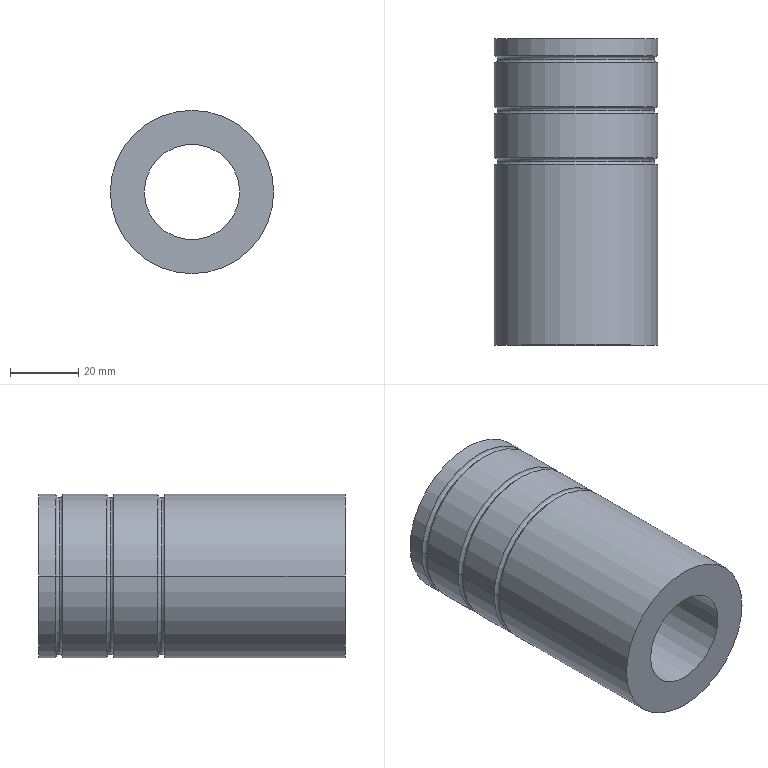Component | SolidWorks | NewDieSet-1_UpperDieSetAssembly-1_GuideBushing-1 | 1 solid | 24 faces | box 48 x 90 x 48 mm | volume 106744 mm3 | torus 12 | cylinder 10 | plane 2 | commonest cylinder face diameters 48 x8 28 x2
build123d program:
from build123d import *

# Parameters (mm, degrees)
SKETCH1_R           = 24
BOSS_EXTRUDE1_DEPTH = 45
SKETCH2_R           = 24
BOSS_EXTRUDE2_DEPTH = 45
SKETCH3_R           = 14
CUT_EXTRUDE1_DEPTH  = 97.187
SKETCH4_R           = 1
LPATTERN1_COUNT     = 3
LPATTERN1_PITCH     = 15


with BuildPart() as part:
    # Sketch1 → Boss-Extrude1 (new body)
    with BuildSketch(Plane.XY):
        with Locations(Location((0, 0, 0), (0, 0, 180))):
            Circle(SKETCH1_R)
    extrude(amount=BOSS_EXTRUDE1_DEPTH)

    # Sketch2 → Boss-Extrude2 (add)
    with BuildSketch(Plane.XY.offset(45)):
        with Locations(Location((0, 0, 0), (0, 0, 180))):
            Circle(SKETCH2_R)
    extrude(amount=BOSS_EXTRUDE2_DEPTH)

    # Sketch3 → Cut-Extrude1 (cut, through all)
    with BuildSketch(Plane.XY.offset(90)):
        Circle(SKETCH3_R)
    extrude(amount=-CUT_EXTRUDE1_DEPTH, mode=Mode.SUBTRACT)

    # Sketch4 → Cut-Revolve1 (revolve, cut)
    with BuildSketch(Plane(origin=(0, 0, 0), x_dir=(1, 0, 0), z_dir=(0, 1, 0)), mode=Mode.PRIVATE) as cut_revolve1_sk:
        with Locations((24, -6)):
            Circle(SKETCH4_R)
    cut_revolve1 = revolve(cut_revolve1_sk.sketch.rotate(Axis((0, 0, 0), (0, 0, 1)), 180), axis=Axis((0, 0, 0), (0, 0, 1)), mode=Mode.SUBTRACT)

    # LPattern1: Cut-Revolve1 ×3
    with Locations(*[(0, 0, i * LPATTERN1_PITCH) for i in range(1, LPATTERN1_COUNT)]):
        add(cut_revolve1, mode=Mode.SUBTRACT)


solid = part.part

# Placed as in the assembly
solid = solid.moved(Location((-216.746, 158.927, 568), (90, 0, 0)))
STEP:
#1=COLOUR_RGB('',0.7922,0.8196,0.9333);
#2=FILL_AREA_STYLE_COLOUR('',#1);
#3=FILL_AREA_STYLE('',(#2));
#4=SURFACE_STYLE_FILL_AREA(#3);
#5=SURFACE_SIDE_STYLE('',(#4));
#6=SURFACE_STYLE_USAGE(.BOTH.,#5);
#7=PRESENTATION_STYLE_ASSIGNMENT((#6));
#8=CARTESIAN_POINT('',(-9.478,4.879,22.362));
#9=VERTEX_POINT('',#8);
#10=CARTESIAN_POINT('',(-9.439,4.84,22.362));
#11=VERTEX_POINT('',#10);
#12=CARTESIAN_POINT('',(-9.478,4.84,22.362));
#13=DIRECTION('',(0.,0.,-1.));
#14=DIRECTION('',(-1.,0.,0.));
#15=AXIS2_PLACEMENT_3D('',#12,#13,#14);
#16=CIRCLE('',#15,0.03937);
#17=EDGE_CURVE('',#9,#11,#16,.T.);
#18=ORIENTED_EDGE('',*,*,#17,.T.);
#19=CARTESIAN_POINT('',(-7.628,4.84,22.362));
#20=VERTEX_POINT('',#19);
#21=CARTESIAN_POINT('',(-8.533,4.84,22.362));
#22=DIRECTION('',(0.,1.,0.));
#23=DIRECTION('',(0.,0.,1.));
#24=AXIS2_PLACEMENT_3D('',#21,#22,#23);
#25=CIRCLE('',#24,0.9055);
#26=EDGE_CURVE('',#11,#20,#25,.T.);
#27=ORIENTED_EDGE('',*,*,#26,.T.);
#28=CARTESIAN_POINT('',(-7.588,4.879,22.362));
#29=VERTEX_POINT('',#28);
#30=CARTESIAN_POINT('',(-7.588,4.84,22.362));
#31=DIRECTION('',(-0.,0.,1.));
#32=DIRECTION('',(1.,0.,0.));
#33=AXIS2_PLACEMENT_3D('',#30,#31,#32);
#34=CIRCLE('',#33,0.03937);
#35=EDGE_CURVE('',#29,#20,#34,.T.);
#36=ORIENTED_EDGE('',*,*,#35,.F.);
#37=CARTESIAN_POINT('',(-8.533,4.879,22.362));
#38=DIRECTION('',(0.,-1.,0.));
#39=DIRECTION('',(1.,0.,0.));
#40=AXIS2_PLACEMENT_3D('',#37,#38,#39);
#41=CIRCLE('',#40,0.9449);
#42=EDGE_CURVE('',#29,#9,#41,.T.);
#43=ORIENTED_EDGE('',*,*,#42,.T.);
#44=EDGE_LOOP('',(#18,#27,#36,#43));
#45=FACE_OUTER_BOUND('',#44,.T.);
#46=CARTESIAN_POINT('',(-8.533,4.84,22.362));
#47=DIRECTION('',(0.,1.,0.));
#48=DIRECTION('',(-1.,0.,0.));
#49=AXIS2_PLACEMENT_3D('',#46,#47,#48);
#50=TOROIDAL_SURFACE('',#49,0.9449,0.03937);
#51=ADVANCED_FACE('',(#45),#50,.F.);
#52=CARTESIAN_POINT('',(-9.478,5.47,22.362));
#53=VERTEX_POINT('',#52);
#54=CARTESIAN_POINT('',(-9.439,5.43,22.362));
#55=VERTEX_POINT('',#54);
#56=CARTESIAN_POINT('',(-9.478,5.43,22.362));
#57=DIRECTION('',(0.,0.,-1.));
#58=DIRECTION('',(-1.,0.,0.));
#59=AXIS2_PLACEMENT_3D('',#56,#57,#58);
#60=CIRCLE('',#59,0.03937);
#61=EDGE_CURVE('',#53,#55,#60,.T.);
#62=ORIENTED_EDGE('',*,*,#61,.T.);
#63=CARTESIAN_POINT('',(-7.628,5.43,22.362));
#64=VERTEX_POINT('',#63);
#65=CARTESIAN_POINT('',(-8.533,5.43,22.362));
#66=DIRECTION('',(0.,1.,0.));
#67=DIRECTION('',(0.,0.,1.));
#68=AXIS2_PLACEMENT_3D('',#65,#66,#67);
#69=CIRCLE('',#68,0.9055);
#70=EDGE_CURVE('',#55,#64,#69,.T.);
#71=ORIENTED_EDGE('',*,*,#70,.T.);
#72=CARTESIAN_POINT('',(-7.588,5.47,22.362));
#73=VERTEX_POINT('',#72);
#74=CARTESIAN_POINT('',(-7.588,5.43,22.362));
#75=DIRECTION('',(-0.,0.,1.));
#76=DIRECTION('',(1.,0.,0.));
#77=AXIS2_PLACEMENT_3D('',#74,#75,#76);
#78=CIRCLE('',#77,0.03937);
#79=EDGE_CURVE('',#73,#64,#78,.T.);
#80=ORIENTED_EDGE('',*,*,#79,.F.);
#81=CARTESIAN_POINT('',(-8.533,5.47,22.362));
#82=DIRECTION('',(0.,-1.,0.));
#83=DIRECTION('',(1.,0.,0.));
#84=AXIS2_PLACEMENT_3D('',#81,#82,#83);
#85=CIRCLE('',#84,0.9449);
#86=EDGE_CURVE('',#73,#53,#85,.T.);
#87=ORIENTED_EDGE('',*,*,#86,.T.);
#88=EDGE_LOOP('',(#62,#71,#80,#87));
#89=FACE_OUTER_BOUND('',#88,.T.);
#90=CARTESIAN_POINT('',(-8.533,5.43,22.362));
#91=DIRECTION('',(0.,1.,0.));
#92=DIRECTION('',(-1.,0.,0.));
#93=AXIS2_PLACEMENT_3D('',#90,#91,#92);
#94=TOROIDAL_SURFACE('',#93,0.9449,0.03937);
#95=ADVANCED_FACE('',(#89),#94,.F.);
#96=CARTESIAN_POINT('',(-9.478,6.06,22.362));
#97=VERTEX_POINT('',#96);
#98=CARTESIAN_POINT('',(-9.439,6.021,22.362));
#99=VERTEX_POINT('',#98);
#100=CARTESIAN_POINT('',(-9.478,6.021,22.362));
#101=DIRECTION('',(0.,0.,-1.));
#102=DIRECTION('',(-1.,0.,0.));
#103=AXIS2_PLACEMENT_3D('',#100,#101,#102);
#104=CIRCLE('',#103,0.03937);
#105=EDGE_CURVE('',#97,#99,#104,.T.);
#106=ORIENTED_EDGE('',*,*,#105,.T.);
#107=CARTESIAN_POINT('',(-7.628,6.021,22.362));
#108=VERTEX_POINT('',#107);
#109=CARTESIAN_POINT('',(-8.533,6.021,22.362));
#110=DIRECTION('',(0.,1.,0.));
#111=DIRECTION('',(0.,0.,1.));
#112=AXIS2_PLACEMENT_3D('',#109,#110,#111);
#113=CIRCLE('',#112,0.9055);
#114=EDGE_CURVE('',#99,#108,#113,.T.);
#115=ORIENTED_EDGE('',*,*,#114,.T.);
#116=CARTESIAN_POINT('',(-7.588,6.06,22.362));
#117=VERTEX_POINT('',#116);
#118=CARTESIAN_POINT('',(-7.588,6.021,22.362));
#119=DIRECTION('',(-0.,0.,1.));
#120=DIRECTION('',(1.,0.,0.));
#121=AXIS2_PLACEMENT_3D('',#118,#119,#120);
#122=CIRCLE('',#121,0.03937);
#123=EDGE_CURVE('',#117,#108,#122,.T.);
#124=ORIENTED_EDGE('',*,*,#123,.F.);
#125=CARTESIAN_POINT('',(-8.533,6.06,22.362));
#126=DIRECTION('',(0.,-1.,0.));
#127=DIRECTION('',(1.,0.,0.));
#128=AXIS2_PLACEMENT_3D('',#125,#126,#127);
#129=CIRCLE('',#128,0.9449);
#130=EDGE_CURVE('',#117,#97,#129,.T.);
#131=ORIENTED_EDGE('',*,*,#130,.T.);
#132=EDGE_LOOP('',(#106,#115,#124,#131));
#133=FACE_OUTER_BOUND('',#132,.T.);
#134=CARTESIAN_POINT('',(-8.533,6.021,22.362));
#135=DIRECTION('',(0.,1.,0.));
#136=DIRECTION('',(-1.,0.,0.));
#137=AXIS2_PLACEMENT_3D('',#134,#135,#136);
#138=TOROIDAL_SURFACE('',#137,0.9449,0.03937);
#139=ADVANCED_FACE('',(#133),#138,.F.);
#140=ORIENTED_EDGE('',*,*,#123,.T.);
#141=CARTESIAN_POINT('',(-8.533,6.021,22.362));
#142=DIRECTION('',(0.,1.,0.));
#143=DIRECTION('',(0.,0.,1.));
#144=AXIS2_PLACEMENT_3D('',#141,#142,#143);
#145=CIRCLE('',#144,0.9055);
#146=EDGE_CURVE('',#108,#99,#145,.T.);
#147=ORIENTED_EDGE('',*,*,#146,.T.);
#148=ORIENTED_EDGE('',*,*,#105,.F.);
#149=CARTESIAN_POINT('',(-8.533,6.06,22.362));
#150=DIRECTION('',(0.,-1.,0.));
#151=DIRECTION('',(1.,0.,0.));
#152=AXIS2_PLACEMENT_3D('',#149,#150,#151);
#153=CIRCLE('',#152,0.9449);
#154=EDGE_CURVE('',#97,#117,#153,.T.);
#155=ORIENTED_EDGE('',*,*,#154,.T.);
#156=EDGE_LOOP('',(#140,#147,#148,#155));
#157=FACE_OUTER_BOUND('',#156,.T.);
#158=CARTESIAN_POINT('',(-8.533,6.021,22.362));
#159=DIRECTION('',(0.,1.,0.));
#160=DIRECTION('',(-1.,0.,0.));
#161=AXIS2_PLACEMENT_3D('',#158,#159,#160);
#162=TOROIDAL_SURFACE('',#161,0.9449,0.03937);
#163=ADVANCED_FACE('',(#157),#162,.F.);
#164=ORIENTED_EDGE('',*,*,#79,.T.);
#165=CARTESIAN_POINT('',(-8.533,5.43,22.362));
#166=DIRECTION('',(0.,1.,0.));
#167=DIRECTION('',(0.,0.,1.));
#168=AXIS2_PLACEMENT_3D('',#165,#166,#167);
#169=CIRCLE('',#168,0.9055);
#170=EDGE_CURVE('',#64,#55,#169,.T.);
#171=ORIENTED_EDGE('',*,*,#170,.T.);
#172=ORIENTED_EDGE('',*,*,#61,.F.);
#173=CARTESIAN_POINT('',(-8.533,5.47,22.362));
#174=DIRECTION('',(0.,-1.,0.));
#175=DIRECTION('',(1.,0.,0.));
#176=AXIS2_PLACEMENT_3D('',#173,#174,#175);
#177=CIRCLE('',#176,0.9449);
#178=EDGE_CURVE('',#53,#73,#177,.T.);
#179=ORIENTED_EDGE('',*,*,#178,.T.);
#180=EDGE_LOOP('',(#164,#171,#172,#179));
#181=FACE_OUTER_BOUND('',#180,.T.);
#182=CARTESIAN_POINT('',(-8.533,5.43,22.362));
#183=DIRECTION('',(0.,1.,0.));
#184=DIRECTION('',(-1.,0.,0.));
#185=AXIS2_PLACEMENT_3D('',#182,#183,#184);
#186=TOROIDAL_SURFACE('',#185,0.9449,0.03937);
#187=ADVANCED_FACE('',(#181),#186,.F.);
#188=ORIENTED_EDGE('',*,*,#35,.T.);
#189=CARTESIAN_POINT('',(-8.533,4.84,22.362));
#190=DIRECTION('',(0.,1.,0.));
#191=DIRECTION('',(0.,0.,1.));
#192=AXIS2_PLACEMENT_3D('',#189,#190,#191);
#193=CIRCLE('',#192,0.9055);
#194=EDGE_CURVE('',#20,#11,#193,.T.);
#195=ORIENTED_EDGE('',*,*,#194,.T.);
#196=ORIENTED_EDGE('',*,*,#17,.F.);
#197=CARTESIAN_POINT('',(-8.533,4.879,22.362));
#198=DIRECTION('',(0.,-1.,0.));
#199=DIRECTION('',(1.,0.,0.));
#200=AXIS2_PLACEMENT_3D('',#197,#198,#199);
#201=CIRCLE('',#200,0.9449);
#202=EDGE_CURVE('',#9,#29,#201,.T.);
#203=ORIENTED_EDGE('',*,*,#202,.T.);
#204=EDGE_LOOP('',(#188,#195,#196,#203));
#205=FACE_OUTER_BOUND('',#204,.T.);
#206=CARTESIAN_POINT('',(-8.533,4.84,22.362));
#207=DIRECTION('',(0.,1.,0.));
#208=DIRECTION('',(-1.,0.,0.));
#209=AXIS2_PLACEMENT_3D('',#206,#207,#208);
#210=TOROIDAL_SURFACE('',#209,0.9449,0.03937);
#211=ADVANCED_FACE('',(#205),#210,.F.);
#212=ORIENTED_EDGE('',*,*,#194,.F.);
#213=CARTESIAN_POINT('',(-7.588,4.8,22.362));
#214=VERTEX_POINT('',#213);
#215=CARTESIAN_POINT('',(-7.588,4.84,22.362));
#216=DIRECTION('',(-0.,0.,1.));
#217=DIRECTION('',(1.,0.,0.));
#218=AXIS2_PLACEMENT_3D('',#215,#216,#217);
#219=CIRCLE('',#218,0.03937);
#220=EDGE_CURVE('',#20,#214,#219,.T.);
#221=ORIENTED_EDGE('',*,*,#220,.T.);
#222=CARTESIAN_POINT('',(-9.478,4.8,22.362));
#223=VERTEX_POINT('',#222);
#224=CARTESIAN_POINT('',(-8.533,4.8,22.362));
#225=DIRECTION('',(0.,1.,0.));
#226=DIRECTION('',(-1.,0.,0.));
#227=AXIS2_PLACEMENT_3D('',#224,#225,#226);
#228=CIRCLE('',#227,0.9449);
#229=EDGE_CURVE('',#214,#223,#228,.T.);
#230=ORIENTED_EDGE('',*,*,#229,.T.);
#231=CARTESIAN_POINT('',(-9.478,4.84,22.362));
#232=DIRECTION('',(0.,0.,-1.));
#233=DIRECTION('',(-1.,0.,0.));
#234=AXIS2_PLACEMENT_3D('',#231,#232,#233);
#235=CIRCLE('',#234,0.03937);
#236=EDGE_CURVE('',#11,#223,#235,.T.);
#237=ORIENTED_EDGE('',*,*,#236,.F.);
#238=EDGE_LOOP('',(#212,#221,#230,#237));
#239=FACE_OUTER_BOUND('',#238,.T.);
#240=CARTESIAN_POINT('',(-8.533,4.84,22.362));
#241=DIRECTION('',(0.,1.,0.));
#242=DIRECTION('',(-1.,0.,0.));
#243=AXIS2_PLACEMENT_3D('',#240,#241,#242);
#244=TOROIDAL_SURFACE('',#243,0.9449,0.03937);
#245=ADVANCED_FACE('',(#239),#244,.F.);
#246=ORIENTED_EDGE('',*,*,#170,.F.);
#247=CARTESIAN_POINT('',(-7.588,5.391,22.362));
#248=VERTEX_POINT('',#247);
#249=CARTESIAN_POINT('',(-7.588,5.43,22.362));
#250=DIRECTION('',(-0.,0.,1.));
#251=DIRECTION('',(1.,0.,0.));
#252=AXIS2_PLACEMENT_3D('',#249,#250,#251);
#253=CIRCLE('',#252,0.03937);
#254=EDGE_CURVE('',#64,#248,#253,.T.);
#255=ORIENTED_EDGE('',*,*,#254,.T.);
#256=CARTESIAN_POINT('',(-9.478,5.391,22.362));
#257=VERTEX_POINT('',#256);
#258=CARTESIAN_POINT('',(-8.533,5.391,22.362));
#259=DIRECTION('',(0.,1.,0.));
#260=DIRECTION('',(-1.,0.,0.));
#261=AXIS2_PLACEMENT_3D('',#258,#259,#260);
#262=CIRCLE('',#261,0.9449);
#263=EDGE_CURVE('',#248,#257,#262,.T.);
#264=ORIENTED_EDGE('',*,*,#263,.T.);
#265=CARTESIAN_POINT('',(-9.478,5.43,22.362));
#266=DIRECTION('',(0.,0.,-1.));
#267=DIRECTION('',(-1.,0.,0.));
#268=AXIS2_PLACEMENT_3D('',#265,#266,#267);
#269=CIRCLE('',#268,0.03937);
#270=EDGE_CURVE('',#55,#257,#269,.T.);
#271=ORIENTED_EDGE('',*,*,#270,.F.);
#272=EDGE_LOOP('',(#246,#255,#264,#271));
#273=FACE_OUTER_BOUND('',#272,.T.);
#274=CARTESIAN_POINT('',(-8.533,5.43,22.362));
#275=DIRECTION('',(0.,1.,0.));
#276=DIRECTION('',(-1.,0.,0.));
#277=AXIS2_PLACEMENT_3D('',#274,#275,#276);
#278=TOROIDAL_SURFACE('',#277,0.9449,0.03937);
#279=ADVANCED_FACE('',(#273),#278,.F.);
#280=ORIENTED_EDGE('',*,*,#146,.F.);
#281=CARTESIAN_POINT('',(-7.588,5.981,22.362));
#282=VERTEX_POINT('',#281);
#283=CARTESIAN_POINT('',(-7.588,6.021,22.362));
#284=DIRECTION('',(-0.,0.,1.));
#285=DIRECTION('',(1.,0.,0.));
#286=AXIS2_PLACEMENT_3D('',#283,#284,#285);
#287=CIRCLE('',#286,0.03937);
#288=EDGE_CURVE('',#108,#282,#287,.T.);
#289=ORIENTED_EDGE('',*,*,#288,.T.);
#290=CARTESIAN_POINT('',(-9.478,5.981,22.362));
#291=VERTEX_POINT('',#290);
#292=CARTESIAN_POINT('',(-8.533,5.981,22.362));
#293=DIRECTION('',(0.,1.,0.));
#294=DIRECTION('',(-1.,0.,0.));
#295=AXIS2_PLACEMENT_3D('',#292,#293,#294);
#296=CIRCLE('',#295,0.9449);
#297=EDGE_CURVE('',#282,#291,#296,.T.);
#298=ORIENTED_EDGE('',*,*,#297,.T.);
#299=CARTESIAN_POINT('',(-9.478,6.021,22.362));
#300=DIRECTION('',(0.,0.,-1.));
#301=DIRECTION('',(-1.,0.,0.));
#302=AXIS2_PLACEMENT_3D('',#299,#300,#301);
#303=CIRCLE('',#302,0.03937);
#304=EDGE_CURVE('',#99,#291,#303,.T.);
#305=ORIENTED_EDGE('',*,*,#304,.F.);
#306=EDGE_LOOP('',(#280,#289,#298,#305));
#307=FACE_OUTER_BOUND('',#306,.T.);
#308=CARTESIAN_POINT('',(-8.533,6.021,22.362));
#309=DIRECTION('',(0.,1.,0.));
#310=DIRECTION('',(-1.,0.,0.));
#311=AXIS2_PLACEMENT_3D('',#308,#309,#310);
#312=TOROIDAL_SURFACE('',#311,0.9449,0.03937);
#313=ADVANCED_FACE('',(#307),#312,.F.);
#314=CARTESIAN_POINT('',(-9.084,6.257,22.362));
#315=VERTEX_POINT('',#314);
#316=CARTESIAN_POINT('',(-7.982,6.257,22.362));
#317=VERTEX_POINT('',#316);
#318=CARTESIAN_POINT('',(-8.533,6.257,22.362));
#319=DIRECTION('',(0.,-1.,0.));
#320=DIRECTION('',(1.,0.,0.));
#321=AXIS2_PLACEMENT_3D('',#318,#319,#320);
#322=CIRCLE('',#321,0.5512);
#323=EDGE_CURVE('',#315,#317,#322,.T.);
#324=ORIENTED_EDGE('',*,*,#323,.F.);
#325=CARTESIAN_POINT('',(-9.084,2.714,22.362));
#326=VERTEX_POINT('',#325);
#327=CARTESIAN_POINT('',(-9.084,6.257,22.362));
#328=DIRECTION('',(0.,-1.,0.));
#329=VECTOR('',#328,39.37);
#330=LINE('',#327,#329);
#331=EDGE_CURVE('',#315,#326,#330,.T.);
#332=ORIENTED_EDGE('',*,*,#331,.T.);
#333=CARTESIAN_POINT('',(-7.982,2.714,22.362));
#334=VERTEX_POINT('',#333);
#335=CARTESIAN_POINT('',(-8.533,2.714,22.362));
#336=DIRECTION('',(0.,-1.,0.));
#337=DIRECTION('',(1.,0.,0.));
#338=AXIS2_PLACEMENT_3D('',#335,#336,#337);
#339=CIRCLE('',#338,0.5512);
#340=EDGE_CURVE('',#326,#334,#339,.T.);
#341=ORIENTED_EDGE('',*,*,#340,.T.);
#342=CARTESIAN_POINT('',(-7.982,6.257,22.362));
#343=DIRECTION('',(0.,-1.,0.));
#344=VECTOR('',#343,39.37);
#345=LINE('',#342,#344);
#346=EDGE_CURVE('',#317,#334,#345,.T.);
#347=ORIENTED_EDGE('',*,*,#346,.F.);
#348=EDGE_LOOP('',(#324,#332,#341,#347));
#349=FACE_OUTER_BOUND('',#348,.T.);
#350=CARTESIAN_POINT('',(-8.533,6.257,22.362));
#351=DIRECTION('',(0.,-1.,0.));
#352=DIRECTION('',(1.,0.,0.));
#353=AXIS2_PLACEMENT_3D('',#350,#351,#352);
#354=CYLINDRICAL_SURFACE('',#353,0.5512);
#355=ADVANCED_FACE('',(#349),#354,.F.);
#356=ORIENTED_EDGE('',*,*,#130,.F.);
#357=CARTESIAN_POINT('',(-7.588,6.257,22.362));
#358=VERTEX_POINT('',#357);
#359=CARTESIAN_POINT('',(-7.588,4.485,22.362));
#360=DIRECTION('',(0.,1.,0.));
#361=VECTOR('',#360,39.37);
#362=LINE('',#359,#361);
#363=EDGE_CURVE('',#117,#358,#362,.T.);
#364=ORIENTED_EDGE('',*,*,#363,.T.);
#365=CARTESIAN_POINT('',(-9.478,6.257,22.362));
#366=VERTEX_POINT('',#365);
#367=CARTESIAN_POINT('',(-8.533,6.257,22.362));
#368=DIRECTION('',(0.,-1.,0.));
#369=DIRECTION('',(1.,0.,0.));
#370=AXIS2_PLACEMENT_3D('',#367,#368,#369);
#371=CIRCLE('',#370,0.9449);
#372=EDGE_CURVE('',#358,#366,#371,.T.);
#373=ORIENTED_EDGE('',*,*,#372,.T.);
#374=CARTESIAN_POINT('',(-9.478,4.485,22.362));
#375=DIRECTION('',(0.,1.,0.));
#376=VECTOR('',#375,39.37);
#377=LINE('',#374,#376);
#378=EDGE_CURVE('',#97,#366,#377,.T.);
#379=ORIENTED_EDGE('',*,*,#378,.F.);
#380=EDGE_LOOP('',(#356,#364,#373,#379));
#381=FACE_OUTER_BOUND('',#380,.T.);
#382=CARTESIAN_POINT('',(-8.533,4.485,22.362));
#383=DIRECTION('',(0.,1.,0.));
#384=DIRECTION('',(-1.,0.,0.));
#385=AXIS2_PLACEMENT_3D('',#382,#383,#384);
#386=CYLINDRICAL_SURFACE('',#385,0.9449);
#387=ADVANCED_FACE('',(#381),#386,.T.);
#388=ORIENTED_EDGE('',*,*,#86,.F.);
#389=CARTESIAN_POINT('',(-7.588,4.485,22.362));
#390=DIRECTION('',(0.,1.,0.));
#391=VECTOR('',#390,39.37);
#392=LINE('',#389,#391);
#393=EDGE_CURVE('',#73,#282,#392,.T.);
#394=ORIENTED_EDGE('',*,*,#393,.T.);
#395=CARTESIAN_POINT('',(-8.533,5.981,22.362));
#396=DIRECTION('',(0.,1.,0.));
#397=DIRECTION('',(-1.,0.,0.));
#398=AXIS2_PLACEMENT_3D('',#395,#396,#397);
#399=CIRCLE('',#398,0.9449);
#400=EDGE_CURVE('',#291,#282,#399,.T.);
#401=ORIENTED_EDGE('',*,*,#400,.F.);
#402=CARTESIAN_POINT('',(-9.478,4.485,22.362));
#403=DIRECTION('',(0.,1.,0.));
#404=VECTOR('',#403,39.37);
#405=LINE('',#402,#404);
#406=EDGE_CURVE('',#53,#291,#405,.T.);
#407=ORIENTED_EDGE('',*,*,#406,.F.);
#408=EDGE_LOOP('',(#388,#394,#401,#407));
#409=FACE_OUTER_BOUND('',#408,.T.);
#410=CARTESIAN_POINT('',(-8.533,4.485,22.362));
#411=DIRECTION('',(0.,1.,0.));
#412=DIRECTION('',(-1.,0.,0.));
#413=AXIS2_PLACEMENT_3D('',#410,#411,#412);
#414=CYLINDRICAL_SURFACE('',#413,0.9449);
#415=ADVANCED_FACE('',(#409),#414,.T.);
#416=CARTESIAN_POINT('',(-7.588,2.714,22.362));
#417=VERTEX_POINT('',#416);
#418=CARTESIAN_POINT('',(-9.478,2.714,22.362));
#419=VERTEX_POINT('',#418);
#420=CARTESIAN_POINT('',(-8.533,2.714,22.362));
#421=DIRECTION('',(0.,-1.,0.));
#422=DIRECTION('',(1.,0.,0.));
#423=AXIS2_PLACEMENT_3D('',#420,#421,#422);
#424=CIRCLE('',#423,0.9449);
#425=EDGE_CURVE('',#417,#419,#424,.T.);
#426=ORIENTED_EDGE('',*,*,#425,.F.);
#427=CARTESIAN_POINT('',(-7.588,4.485,22.362));
#428=DIRECTION('',(0.,1.,0.));
#429=VECTOR('',#428,39.37);
#430=LINE('',#427,#429);
#431=EDGE_CURVE('',#417,#214,#430,.T.);
#432=ORIENTED_EDGE('',*,*,#431,.T.);
#433=CARTESIAN_POINT('',(-8.533,4.8,22.362));
#434=DIRECTION('',(0.,1.,0.));
#435=DIRECTION('',(-1.,0.,0.));
#436=AXIS2_PLACEMENT_3D('',#433,#434,#435);
#437=CIRCLE('',#436,0.9449);
#438=EDGE_CURVE('',#223,#214,#437,.T.);
#439=ORIENTED_EDGE('',*,*,#438,.F.);
#440=CARTESIAN_POINT('',(-9.478,4.485,22.362));
#441=DIRECTION('',(0.,1.,0.));
#442=VECTOR('',#441,39.37);
#443=LINE('',#440,#442);
#444=EDGE_CURVE('',#419,#223,#443,.T.);
#445=ORIENTED_EDGE('',*,*,#444,.F.);
#446=EDGE_LOOP('',(#426,#432,#439,#445));
#447=FACE_OUTER_BOUND('',#446,.T.);
#448=CARTESIAN_POINT('',(-8.533,4.485,22.362));
#449=DIRECTION('',(0.,1.,0.));
#450=DIRECTION('',(-1.,0.,0.));
#451=AXIS2_PLACEMENT_3D('',#448,#449,#450);
#452=CYLINDRICAL_SURFACE('',#451,0.9449);
#453=ADVANCED_FACE('',(#447),#452,.T.);
#454=ORIENTED_EDGE('',*,*,#42,.F.);
#455=CARTESIAN_POINT('',(-7.588,4.485,22.362));
#456=DIRECTION('',(0.,1.,0.));
#457=VECTOR('',#456,39.37);
#458=LINE('',#455,#457);
#459=EDGE_CURVE('',#29,#248,#458,.T.);
#460=ORIENTED_EDGE('',*,*,#459,.T.);
#461=CARTESIAN_POINT('',(-8.533,5.391,22.362));
#462=DIRECTION('',(0.,1.,0.));
#463=DIRECTION('',(-1.,0.,0.));
#464=AXIS2_PLACEMENT_3D('',#461,#462,#463);
#465=CIRCLE('',#464,0.9449);
#466=EDGE_CURVE('',#257,#248,#465,.T.);
#467=ORIENTED_EDGE('',*,*,#466,.F.);
#468=CARTESIAN_POINT('',(-9.478,4.485,22.362));
#469=DIRECTION('',(0.,1.,0.));
#470=VECTOR('',#469,39.37);
#471=LINE('',#468,#470);
#472=EDGE_CURVE('',#9,#257,#471,.T.);
#473=ORIENTED_EDGE('',*,*,#472,.F.);
#474=EDGE_LOOP('',(#454,#460,#467,#473));
#475=FACE_OUTER_BOUND('',#474,.T.);
#476=CARTESIAN_POINT('',(-8.533,4.485,22.362));
#477=DIRECTION('',(0.,1.,0.));
#478=DIRECTION('',(-1.,0.,0.));
#479=AXIS2_PLACEMENT_3D('',#476,#477,#478);
#480=CYLINDRICAL_SURFACE('',#479,0.9449);
#481=ADVANCED_FACE('',(#475),#480,.T.);
#482=ORIENTED_EDGE('',*,*,#459,.F.);
#483=ORIENTED_EDGE('',*,*,#202,.F.);
#484=ORIENTED_EDGE('',*,*,#472,.T.);
#485=ORIENTED_EDGE('',*,*,#263,.F.);
#486=EDGE_LOOP('',(#482,#483,#484,#485));
#487=FACE_OUTER_BOUND('',#486,.T.);
#488=CARTESIAN_POINT('',(-8.533,4.485,22.362));
#489=DIRECTION('',(0.,1.,0.));
#490=DIRECTION('',(-1.,0.,0.));
#491=AXIS2_PLACEMENT_3D('',#488,#489,#490);
#492=CYLINDRICAL_SURFACE('',#491,0.9449);
#493=ADVANCED_FACE('',(#487),#492,.T.);
#494=ORIENTED_EDGE('',*,*,#431,.F.);
#495=CARTESIAN_POINT('',(-8.533,2.714,22.362));
#496=DIRECTION('',(0.,-1.,0.));
#497=DIRECTION('',(1.,0.,0.));
#498=AXIS2_PLACEMENT_3D('',#495,#496,#497);
#499=CIRCLE('',#498,0.9449);
#500=EDGE_CURVE('',#419,#417,#499,.T.);
#501=ORIENTED_EDGE('',*,*,#500,.F.);
#502=ORIENTED_EDGE('',*,*,#444,.T.);
#503=ORIENTED_EDGE('',*,*,#229,.F.);
#504=EDGE_LOOP('',(#494,#501,#502,#503));
#505=FACE_OUTER_BOUND('',#504,.T.);
#506=CARTESIAN_POINT('',(-8.533,4.485,22.362));
#507=DIRECTION('',(0.,1.,0.));
#508=DIRECTION('',(-1.,0.,0.));
#509=AXIS2_PLACEMENT_3D('',#506,#507,#508);
#510=CYLINDRICAL_SURFACE('',#509,0.9449);
#511=ADVANCED_FACE('',(#505),#510,.T.);
#512=ORIENTED_EDGE('',*,*,#393,.F.);
#513=ORIENTED_EDGE('',*,*,#178,.F.);
#514=ORIENTED_EDGE('',*,*,#406,.T.);
#515=ORIENTED_EDGE('',*,*,#297,.F.);
#516=EDGE_LOOP('',(#512,#513,#514,#515));
#517=FACE_OUTER_BOUND('',#516,.T.);
#518=CARTESIAN_POINT('',(-8.533,4.485,22.362));
#519=DIRECTION('',(0.,1.,0.));
#520=DIRECTION('',(-1.,0.,0.));
#521=AXIS2_PLACEMENT_3D('',#518,#519,#520);
#522=CYLINDRICAL_SURFACE('',#521,0.9449);
#523=ADVANCED_FACE('',(#517),#522,.T.);
#524=ORIENTED_EDGE('',*,*,#363,.F.);
#525=ORIENTED_EDGE('',*,*,#154,.F.);
#526=ORIENTED_EDGE('',*,*,#378,.T.);
#527=CARTESIAN_POINT('',(-8.533,6.257,22.362));
#528=DIRECTION('',(0.,-1.,0.));
#529=DIRECTION('',(1.,0.,0.));
#530=AXIS2_PLACEMENT_3D('',#527,#528,#529);
#531=CIRCLE('',#530,0.9449);
#532=EDGE_CURVE('',#366,#358,#531,.T.);
#533=ORIENTED_EDGE('',*,*,#532,.T.);
#534=EDGE_LOOP('',(#524,#525,#526,#533));
#535=FACE_OUTER_BOUND('',#534,.T.);
#536=CARTESIAN_POINT('',(-8.533,4.485,22.362));
#537=DIRECTION('',(0.,1.,0.));
#538=DIRECTION('',(-1.,0.,0.));
#539=AXIS2_PLACEMENT_3D('',#536,#537,#538);
#540=CYLINDRICAL_SURFACE('',#539,0.9449);
#541=ADVANCED_FACE('',(#535),#540,.T.);
#542=CARTESIAN_POINT('',(-8.533,6.257,22.362));
#543=DIRECTION('',(0.,-1.,0.));
#544=DIRECTION('',(1.,0.,0.));
#545=AXIS2_PLACEMENT_3D('',#542,#543,#544);
#546=CIRCLE('',#545,0.5512);
#547=EDGE_CURVE('',#317,#315,#546,.T.);
#548=ORIENTED_EDGE('',*,*,#547,.T.);
#549=ORIENTED_EDGE('',*,*,#323,.T.);
#550=EDGE_LOOP('',(#548,#549));
#551=FACE_BOUND('',#550,.T.);
#552=ORIENTED_EDGE('',*,*,#532,.F.);
#553=ORIENTED_EDGE('',*,*,#372,.F.);
#554=EDGE_LOOP('',(#552,#553));
#555=FACE_OUTER_BOUND('',#554,.T.);
#556=CARTESIAN_POINT('',(-8.533,6.257,22.362));
#557=DIRECTION('',(0.,-1.,0.));
#558=DIRECTION('',(1.,0.,0.));
#559=AXIS2_PLACEMENT_3D('',#556,#557,#558);
#560=PLANE('',#559);
#561=ADVANCED_FACE('',(#551,#555),#560,.F.);
#562=CARTESIAN_POINT('',(-8.533,2.714,22.362));
#563=DIRECTION('',(0.,-1.,0.));
#564=DIRECTION('',(1.,0.,0.));
#565=AXIS2_PLACEMENT_3D('',#562,#563,#564);
#566=CIRCLE('',#565,0.5512);
#567=EDGE_CURVE('',#334,#326,#566,.T.);
#568=ORIENTED_EDGE('',*,*,#567,.F.);
#569=ORIENTED_EDGE('',*,*,#340,.F.);
#570=EDGE_LOOP('',(#568,#569));
#571=FACE_BOUND('',#570,.T.);
#572=ORIENTED_EDGE('',*,*,#500,.T.);
#573=ORIENTED_EDGE('',*,*,#425,.T.);
#574=EDGE_LOOP('',(#572,#573));
#575=FACE_OUTER_BOUND('',#574,.T.);
#576=CARTESIAN_POINT('',(-8.533,2.714,22.362));
#577=DIRECTION('',(0.,-1.,0.));
#578=DIRECTION('',(1.,0.,0.));
#579=AXIS2_PLACEMENT_3D('',#576,#577,#578);
#580=PLANE('',#579);
#581=ADVANCED_FACE('',(#571,#575),#580,.T.);
#582=ORIENTED_EDGE('',*,*,#331,.F.);
#583=ORIENTED_EDGE('',*,*,#547,.F.);
#584=ORIENTED_EDGE('',*,*,#346,.T.);
#585=ORIENTED_EDGE('',*,*,#567,.T.);
#586=EDGE_LOOP('',(#582,#583,#584,#585));
#587=FACE_OUTER_BOUND('',#586,.T.);
#588=CARTESIAN_POINT('',(-8.533,6.257,22.362));
#589=DIRECTION('',(0.,-1.,0.));
#590=DIRECTION('',(1.,0.,0.));
#591=AXIS2_PLACEMENT_3D('',#588,#589,#590);
#592=CYLINDRICAL_SURFACE('',#591,0.5512);
#593=ADVANCED_FACE('',(#587),#592,.F.);
#594=ORIENTED_EDGE('',*,*,#114,.F.);
#595=ORIENTED_EDGE('',*,*,#304,.T.);
#596=ORIENTED_EDGE('',*,*,#400,.T.);
#597=ORIENTED_EDGE('',*,*,#288,.F.);
#598=EDGE_LOOP('',(#594,#595,#596,#597));
#599=FACE_OUTER_BOUND('',#598,.T.);
#600=CARTESIAN_POINT('',(-8.533,6.021,22.362));
#601=DIRECTION('',(0.,1.,0.));
#602=DIRECTION('',(-1.,0.,0.));
#603=AXIS2_PLACEMENT_3D('',#600,#601,#602);
#604=TOROIDAL_SURFACE('',#603,0.9449,0.03937);
#605=ADVANCED_FACE('',(#599),#604,.F.);
#606=ORIENTED_EDGE('',*,*,#70,.F.);
#607=ORIENTED_EDGE('',*,*,#270,.T.);
#608=ORIENTED_EDGE('',*,*,#466,.T.);
#609=ORIENTED_EDGE('',*,*,#254,.F.);
#610=EDGE_LOOP('',(#606,#607,#608,#609));
#611=FACE_OUTER_BOUND('',#610,.T.);
#612=CARTESIAN_POINT('',(-8.533,5.43,22.362));
#613=DIRECTION('',(0.,1.,0.));
#614=DIRECTION('',(-1.,0.,0.));
#615=AXIS2_PLACEMENT_3D('',#612,#613,#614);
#616=TOROIDAL_SURFACE('',#615,0.9449,0.03937);
#617=ADVANCED_FACE('',(#611),#616,.F.);
#618=ORIENTED_EDGE('',*,*,#26,.F.);
#619=ORIENTED_EDGE('',*,*,#236,.T.);
#620=ORIENTED_EDGE('',*,*,#438,.T.);
#621=ORIENTED_EDGE('',*,*,#220,.F.);
#622=EDGE_LOOP('',(#618,#619,#620,#621));
#623=FACE_OUTER_BOUND('',#622,.T.);
#624=CARTESIAN_POINT('',(-8.533,4.84,22.362));
#625=DIRECTION('',(0.,1.,0.));
#626=DIRECTION('',(-1.,0.,0.));
#627=AXIS2_PLACEMENT_3D('',#624,#625,#626);
#628=TOROIDAL_SURFACE('',#627,0.9449,0.03937);
#629=ADVANCED_FACE('',(#623),#628,.F.);
#630=CLOSED_SHELL('',(#51,#95,#139,#163,#187,#211,#245,#279,#313,#355,#387,#415,#453,#481,#493,#511,#523,#541,#561,#581,#593,#605,#617,#629));
#631=MANIFOLD_SOLID_BREP('',#630);
#632=STYLED_ITEM('',(#7),#631);
#633=PRESENTATION_LAYER_ASSIGNMENT('','',(#632));
#634=CARTESIAN_POINT('',(0.,0.,0.));
#635=DIRECTION('',(0.,0.,1.));
#636=DIRECTION('',(1.,0.,0.));
#637=AXIS2_PLACEMENT_3D('',#634,#635,#636);
#638=(LENGTH_UNIT()NAMED_UNIT(*)SI_UNIT($,.METRE.));
#639=LENGTH_MEASURE_WITH_UNIT(LENGTH_MEASURE(0.0254),#638);
#640=DIMENSIONAL_EXPONENTS(1.,0.,0.,0.,0.,0.,0.);
#641=(CONVERSION_BASED_UNIT('',#639)LENGTH_UNIT()NAMED_UNIT(#640));
#642=UNCERTAINTY_MEASURE_WITH_UNIT(LENGTH_MEASURE(0.00001),#641,'','');
#643=(NAMED_UNIT(*)PLANE_ANGLE_UNIT()SI_UNIT($,.RADIAN.));
#644=(NAMED_UNIT(*)SI_UNIT($,.STERADIAN.)SOLID_ANGLE_UNIT());
#645=(GEOMETRIC_REPRESENTATION_CONTEXT(3)GLOBAL_UNCERTAINTY_ASSIGNED_CONTEXT((#642))GLOBAL_UNIT_ASSIGNED_CONTEXT((#641,#643,#644))REPRESENTATION_CONTEXT('',''));
#646=ADVANCED_BREP_SHAPE_REPRESENTATION('',(#631,#637),#645);
#647=(LENGTH_UNIT()NAMED_UNIT(*)SI_UNIT($,.METRE.));
#648=LENGTH_MEASURE_WITH_UNIT(LENGTH_MEASURE(0.0254),#647);
#649=DIMENSIONAL_EXPONENTS(1.,0.,0.,0.,0.,0.,0.);
#650=(CONVERSION_BASED_UNIT('',#648)LENGTH_UNIT()NAMED_UNIT(#649));
#651=UNCERTAINTY_MEASURE_WITH_UNIT(LENGTH_MEASURE(0.00001),#650,'','');
#652=(NAMED_UNIT(*)PLANE_ANGLE_UNIT()SI_UNIT($,.RADIAN.));
#653=(NAMED_UNIT(*)SI_UNIT($,.STERADIAN.)SOLID_ANGLE_UNIT());
#654=(GEOMETRIC_REPRESENTATION_CONTEXT(3)GLOBAL_UNCERTAINTY_ASSIGNED_CONTEXT((#651))GLOBAL_UNIT_ASSIGNED_CONTEXT((#650,#652,#653))REPRESENTATION_CONTEXT('',''));
#655=MECHANICAL_DESIGN_GEOMETRIC_PRESENTATION_REPRESENTATION('',(#632),#654);